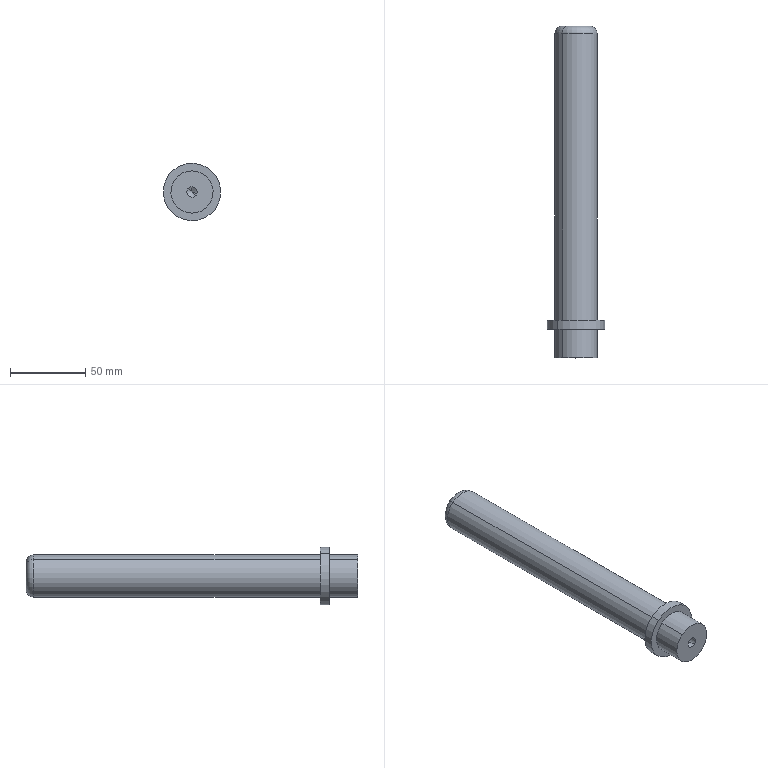Component | SolidWorks | NewDieSet-1_LowerDieSetAssembly-1_GuidePin-2 | 1 solid | 16 faces | box 38 x 220 x 38 mm | volume 137309 mm3 | cylinder 8 | plane 4 | cone 2 | torus 2 | commonest cylinder face diameters 28 x4 6.8 x2 38 x2
build123d program:
from build123d import *

# Parameters (mm, degrees)
SKETCH1_R             = 14
BOSS_EXTRUDE1_DEPTH   = 220
FILLET1_R             = 5
SKETCH4_R             = 19
BOSS_EXTRUDE2_DEPTH   = 6
M8_TAPPED_HOLE1_D     = 6.8
M8_TAPPED_HOLE1_DEPTH = 22.25
M8_TAPPED_HOLE1_TIP   = 2.043


with BuildPart() as part:
    # Sketch1 → Boss-Extrude1 (new body)
    with BuildSketch(Plane.XY):
        Circle(SKETCH1_R)
    extrude(amount=BOSS_EXTRUDE1_DEPTH)

    # Fillet1
    fillet1_edges = [part.edges().sort_by_distance(p)[0] for p in [
        (-14, 0, 0),
    ]]
    fillet(fillet1_edges, radius=FILLET1_R)

    # Sketch4 → Boss-Extrude2 (add)
    with BuildSketch(Plane.XY.offset(201)):
        Circle(SKETCH4_R)
    extrude(amount=-BOSS_EXTRUDE2_DEPTH)

    # M8 Tapped Hole1
    with Locations(Plane.XY.offset(220)):
        with Locations((0, 0)):
            Hole(M8_TAPPED_HOLE1_D / 2, depth=M8_TAPPED_HOLE1_DEPTH)
            with Locations((0, 0, -(M8_TAPPED_HOLE1_DEPTH + M8_TAPPED_HOLE1_TIP / 2))):  # 118° drill point
                Cone(0, M8_TAPPED_HOLE1_D / 2, M8_TAPPED_HOLE1_TIP, mode=Mode.SUBTRACT)


solid = part.part

# Placed as in the assembly
solid = solid.moved(Location((-181.746, 198.927, 138), (90, 0, 0)))
STEP:
#1=COLOUR_RGB('',0.7922,0.8196,0.9333);
#2=FILL_AREA_STYLE_COLOUR('',#1);
#3=FILL_AREA_STYLE('',(#2));
#4=SURFACE_STYLE_FILL_AREA(#3);
#5=SURFACE_SIDE_STYLE('',(#4));
#6=SURFACE_STYLE_USAGE(.BOTH.,#5);
#7=PRESENTATION_STYLE_ASSIGNMENT((#6));
#8=CARTESIAN_POINT('',(-7.241,0.04634,5.536));
#9=VERTEX_POINT('',#8);
#10=CARTESIAN_POINT('',(-7.07,0.04634,5.33));
#11=VERTEX_POINT('',#10);
#12=CARTESIAN_POINT('',(-7.155,0.04634,5.433));
#13=DIRECTION('',(0.,-1.,0.));
#14=DIRECTION('',(0.6389,0.,-0.7693));
#15=AXIS2_PLACEMENT_3D('',#12,#13,#14);
#16=CIRCLE('',#15,0.1339);
#17=EDGE_CURVE('',#9,#11,#16,.T.);
#18=ORIENTED_EDGE('',*,*,#17,.F.);
#19=CARTESIAN_POINT('',(-7.241,-0.8296,5.536));
#20=VERTEX_POINT('',#19);
#21=CARTESIAN_POINT('',(-7.241,-0.8296,5.536));
#22=DIRECTION('',(0.,-1.,0.));
#23=VECTOR('',#22,39.37);
#24=LINE('',#21,#23);
#25=EDGE_CURVE('',#9,#20,#24,.T.);
#26=ORIENTED_EDGE('',*,*,#25,.T.);
#27=CARTESIAN_POINT('',(-7.07,-0.8296,5.33));
#28=VERTEX_POINT('',#27);
#29=CARTESIAN_POINT('',(-7.155,-0.8296,5.433));
#30=DIRECTION('',(0.,-1.,0.));
#31=DIRECTION('',(0.6389,0.,-0.7693));
#32=AXIS2_PLACEMENT_3D('',#29,#30,#31);
#33=CIRCLE('',#32,0.1339);
#34=EDGE_CURVE('',#20,#28,#33,.T.);
#35=ORIENTED_EDGE('',*,*,#34,.T.);
#36=CARTESIAN_POINT('',(-7.07,-0.8296,5.33));
#37=DIRECTION('',(0.,-1.,0.));
#38=VECTOR('',#37,39.37);
#39=LINE('',#36,#38);
#40=EDGE_CURVE('',#11,#28,#39,.T.);
#41=ORIENTED_EDGE('',*,*,#40,.F.);
#42=EDGE_LOOP('',(#18,#26,#35,#41));
#43=FACE_OUTER_BOUND('',#42,.T.);
#44=CARTESIAN_POINT('',(-7.155,-0.8296,5.433));
#45=DIRECTION('',(0.,-1.,0.));
#46=DIRECTION('',(0.6389,0.,-0.7693));
#47=AXIS2_PLACEMENT_3D('',#44,#45,#46);
#48=CYLINDRICAL_SURFACE('',#47,0.1339);
#49=ADVANCED_FACE('',(#43),#48,.F.);
#50=CARTESIAN_POINT('',(-7.155,0.1268,5.433));
#51=VERTEX_POINT('',#50);
#52=CARTESIAN_POINT('',(-7.07,0.04634,5.33));
#53=DIRECTION('',(0.5476,-0.515,-0.6594));
#54=VECTOR('',#53,39.37);
#55=LINE('',#52,#54);
#56=EDGE_CURVE('',#51,#11,#55,.T.);
#57=ORIENTED_EDGE('',*,*,#56,.F.);
#58=CARTESIAN_POINT('',(-7.241,0.04634,5.536));
#59=DIRECTION('',(-0.5476,-0.515,0.6594));
#60=VECTOR('',#59,39.37);
#61=LINE('',#58,#60);
#62=EDGE_CURVE('',#51,#9,#61,.T.);
#63=ORIENTED_EDGE('',*,*,#62,.T.);
#64=ORIENTED_EDGE('',*,*,#17,.T.);
#65=EDGE_LOOP('',(#57,#63,#64));
#66=FACE_OUTER_BOUND('',#65,.T.);
#67=CARTESIAN_POINT('',(-7.155,0.04634,5.433));
#68=DIRECTION('',(0.,-1.,0.));
#69=DIRECTION('',(0.6389,0.,-0.7693));
#70=AXIS2_PLACEMENT_3D('',#67,#68,#69);
#71=CONICAL_SURFACE('',#70,0.1339,1.03);
#72=ADVANCED_FACE('',(#66),#71,.F.);
#73=CARTESIAN_POINT('',(-6.803,-0.8296,5.009));
#74=VERTEX_POINT('',#73);
#75=CARTESIAN_POINT('',(-7.508,-0.8296,5.857));
#76=VERTEX_POINT('',#75);
#77=CARTESIAN_POINT('',(-7.155,-0.8296,5.433));
#78=DIRECTION('',(0.,-1.,0.));
#79=DIRECTION('',(0.6389,0.,-0.7693));
#80=AXIS2_PLACEMENT_3D('',#77,#78,#79);
#81=CIRCLE('',#80,0.5512);
#82=EDGE_CURVE('',#74,#76,#81,.T.);
#83=ORIENTED_EDGE('',*,*,#82,.F.);
#84=CARTESIAN_POINT('',(-6.803,-0.08161,5.009));
#85=VERTEX_POINT('',#84);
#86=CARTESIAN_POINT('',(-6.803,-0.8296,5.009));
#87=DIRECTION('',(0.,1.,0.));
#88=VECTOR('',#87,39.37);
#89=LINE('',#86,#88);
#90=EDGE_CURVE('',#74,#85,#89,.T.);
#91=ORIENTED_EDGE('',*,*,#90,.T.);
#92=CARTESIAN_POINT('',(-7.508,-0.08161,5.857));
#93=VERTEX_POINT('',#92);
#94=CARTESIAN_POINT('',(-7.155,-0.08161,5.433));
#95=DIRECTION('',(0.,-1.,0.));
#96=DIRECTION('',(0.6389,0.,-0.7693));
#97=AXIS2_PLACEMENT_3D('',#94,#95,#96);
#98=CIRCLE('',#97,0.5512);
#99=EDGE_CURVE('',#85,#93,#98,.T.);
#100=ORIENTED_EDGE('',*,*,#99,.T.);
#101=CARTESIAN_POINT('',(-7.508,-0.8296,5.857));
#102=DIRECTION('',(0.,1.,0.));
#103=VECTOR('',#102,39.37);
#104=LINE('',#101,#103);
#105=EDGE_CURVE('',#76,#93,#104,.T.);
#106=ORIENTED_EDGE('',*,*,#105,.F.);
#107=EDGE_LOOP('',(#83,#91,#100,#106));
#108=FACE_OUTER_BOUND('',#107,.T.);
#109=CARTESIAN_POINT('',(-7.155,-0.8296,5.433));
#110=DIRECTION('',(0.,1.,0.));
#111=DIRECTION('',(-0.6389,0.,0.7693));
#112=AXIS2_PLACEMENT_3D('',#109,#110,#111);
#113=CYLINDRICAL_SURFACE('',#112,0.5512);
#114=ADVANCED_FACE('',(#108),#113,.T.);
#115=CARTESIAN_POINT('',(-6.677,0.1546,4.858));
#116=VERTEX_POINT('',#115);
#117=CARTESIAN_POINT('',(-7.633,0.1546,6.009));
#118=VERTEX_POINT('',#117);
#119=CARTESIAN_POINT('',(-7.155,0.1546,5.433));
#120=DIRECTION('',(0.,-1.,0.));
#121=DIRECTION('',(0.6389,0.,-0.7693));
#122=AXIS2_PLACEMENT_3D('',#119,#120,#121);
#123=CIRCLE('',#122,0.748);
#124=EDGE_CURVE('',#116,#118,#123,.T.);
#125=ORIENTED_EDGE('',*,*,#124,.T.);
#126=CARTESIAN_POINT('',(-7.633,-0.08161,6.009));
#127=VERTEX_POINT('',#126);
#128=CARTESIAN_POINT('',(-7.633,0.1546,6.009));
#129=DIRECTION('',(0.,-1.,0.));
#130=VECTOR('',#129,39.37);
#131=LINE('',#128,#130);
#132=EDGE_CURVE('',#118,#127,#131,.T.);
#133=ORIENTED_EDGE('',*,*,#132,.T.);
#134=CARTESIAN_POINT('',(-6.677,-0.08161,4.858));
#135=VERTEX_POINT('',#134);
#136=CARTESIAN_POINT('',(-7.155,-0.08161,5.433));
#137=DIRECTION('',(0.,-1.,0.));
#138=DIRECTION('',(0.6389,0.,-0.7693));
#139=AXIS2_PLACEMENT_3D('',#136,#137,#138);
#140=CIRCLE('',#139,0.748);
#141=EDGE_CURVE('',#135,#127,#140,.T.);
#142=ORIENTED_EDGE('',*,*,#141,.F.);
#143=CARTESIAN_POINT('',(-6.677,0.1546,4.858));
#144=DIRECTION('',(0.,-1.,0.));
#145=VECTOR('',#144,39.37);
#146=LINE('',#143,#145);
#147=EDGE_CURVE('',#116,#135,#146,.T.);
#148=ORIENTED_EDGE('',*,*,#147,.F.);
#149=EDGE_LOOP('',(#125,#133,#142,#148));
#150=FACE_OUTER_BOUND('',#149,.T.);
#151=CARTESIAN_POINT('',(-7.155,0.1546,5.433));
#152=DIRECTION('',(0.,-1.,0.));
#153=DIRECTION('',(0.6389,0.,-0.7693));
#154=AXIS2_PLACEMENT_3D('',#151,#152,#153);
#155=CYLINDRICAL_SURFACE('',#154,0.748);
#156=ADVANCED_FACE('',(#150),#155,.T.);
#157=CARTESIAN_POINT('',(-7.382,7.832,5.706));
#158=VERTEX_POINT('',#157);
#159=CARTESIAN_POINT('',(-6.929,7.832,5.16));
#160=VERTEX_POINT('',#159);
#161=CARTESIAN_POINT('',(-7.155,7.832,5.433));
#162=DIRECTION('',(0.,1.,0.));
#163=DIRECTION('',(0.6389,0.,-0.7693));
#164=AXIS2_PLACEMENT_3D('',#161,#162,#163);
#165=CIRCLE('',#164,0.3543);
#166=EDGE_CURVE('',#158,#160,#165,.T.);
#167=ORIENTED_EDGE('',*,*,#166,.F.);
#168=CARTESIAN_POINT('',(-7.508,7.635,5.857));
#169=VERTEX_POINT('',#168);
#170=CARTESIAN_POINT('',(-7.382,7.635,5.706));
#171=DIRECTION('',(0.7693,0.,0.6389));
#172=DIRECTION('',(0.6389,0.,-0.7693));
#173=AXIS2_PLACEMENT_3D('',#170,#171,#172);
#174=CIRCLE('',#173,0.1969);
#175=EDGE_CURVE('',#158,#169,#174,.T.);
#176=ORIENTED_EDGE('',*,*,#175,.T.);
#177=CARTESIAN_POINT('',(-6.803,7.635,5.009));
#178=VERTEX_POINT('',#177);
#179=CARTESIAN_POINT('',(-7.155,7.635,5.433));
#180=DIRECTION('',(0.,-1.,0.));
#181=DIRECTION('',(0.6389,0.,-0.7693));
#182=AXIS2_PLACEMENT_3D('',#179,#180,#181);
#183=CIRCLE('',#182,0.5512);
#184=EDGE_CURVE('',#178,#169,#183,.T.);
#185=ORIENTED_EDGE('',*,*,#184,.F.);
#186=CARTESIAN_POINT('',(-6.929,7.635,5.16));
#187=DIRECTION('',(-0.7693,0.,-0.6389));
#188=DIRECTION('',(-0.6389,0.,0.7693));
#189=AXIS2_PLACEMENT_3D('',#186,#187,#188);
#190=CIRCLE('',#189,0.1969);
#191=EDGE_CURVE('',#160,#178,#190,.T.);
#192=ORIENTED_EDGE('',*,*,#191,.F.);
#193=EDGE_LOOP('',(#167,#176,#185,#192));
#194=FACE_OUTER_BOUND('',#193,.T.);
#195=CARTESIAN_POINT('',(-7.155,7.635,5.433));
#196=DIRECTION('',(0.,-1.,0.));
#197=DIRECTION('',(0.6389,0.,-0.7693));
#198=AXIS2_PLACEMENT_3D('',#195,#196,#197);
#199=TOROIDAL_SURFACE('',#198,0.3543,0.1969);
#200=ADVANCED_FACE('',(#194),#199,.T.);
#201=CARTESIAN_POINT('',(-6.803,0.1546,5.009));
#202=VERTEX_POINT('',#201);
#203=CARTESIAN_POINT('',(-7.508,0.1546,5.857));
#204=VERTEX_POINT('',#203);
#205=CARTESIAN_POINT('',(-7.155,0.1546,5.433));
#206=DIRECTION('',(0.,-1.,0.));
#207=DIRECTION('',(0.6389,0.,-0.7693));
#208=AXIS2_PLACEMENT_3D('',#205,#206,#207);
#209=CIRCLE('',#208,0.5512);
#210=EDGE_CURVE('',#202,#204,#209,.T.);
#211=ORIENTED_EDGE('',*,*,#210,.F.);
#212=CARTESIAN_POINT('',(-6.803,-0.8296,5.009));
#213=DIRECTION('',(0.,1.,0.));
#214=VECTOR('',#213,39.37);
#215=LINE('',#212,#214);
#216=EDGE_CURVE('',#202,#178,#215,.T.);
#217=ORIENTED_EDGE('',*,*,#216,.T.);
#218=ORIENTED_EDGE('',*,*,#184,.T.);
#219=CARTESIAN_POINT('',(-7.508,-0.8296,5.857));
#220=DIRECTION('',(0.,1.,0.));
#221=VECTOR('',#220,39.37);
#222=LINE('',#219,#221);
#223=EDGE_CURVE('',#204,#169,#222,.T.);
#224=ORIENTED_EDGE('',*,*,#223,.F.);
#225=EDGE_LOOP('',(#211,#217,#218,#224));
#226=FACE_OUTER_BOUND('',#225,.T.);
#227=CARTESIAN_POINT('',(-7.155,-0.8296,5.433));
#228=DIRECTION('',(0.,1.,0.));
#229=DIRECTION('',(-0.6389,0.,0.7693));
#230=AXIS2_PLACEMENT_3D('',#227,#228,#229);
#231=CYLINDRICAL_SURFACE('',#230,0.5512);
#232=ADVANCED_FACE('',(#226),#231,.T.);
#233=ORIENTED_EDGE('',*,*,#216,.F.);
#234=CARTESIAN_POINT('',(-7.155,0.1546,5.433));
#235=DIRECTION('',(0.,-1.,0.));
#236=DIRECTION('',(0.6389,0.,-0.7693));
#237=AXIS2_PLACEMENT_3D('',#234,#235,#236);
#238=CIRCLE('',#237,0.5512);
#239=EDGE_CURVE('',#204,#202,#238,.T.);
#240=ORIENTED_EDGE('',*,*,#239,.F.);
#241=ORIENTED_EDGE('',*,*,#223,.T.);
#242=CARTESIAN_POINT('',(-7.155,7.635,5.433));
#243=DIRECTION('',(0.,-1.,0.));
#244=DIRECTION('',(0.6389,0.,-0.7693));
#245=AXIS2_PLACEMENT_3D('',#242,#243,#244);
#246=CIRCLE('',#245,0.5512);
#247=EDGE_CURVE('',#169,#178,#246,.T.);
#248=ORIENTED_EDGE('',*,*,#247,.T.);
#249=EDGE_LOOP('',(#233,#240,#241,#248));
#250=FACE_OUTER_BOUND('',#249,.T.);
#251=CARTESIAN_POINT('',(-7.155,-0.8296,5.433));
#252=DIRECTION('',(0.,1.,0.));
#253=DIRECTION('',(-0.6389,0.,0.7693));
#254=AXIS2_PLACEMENT_3D('',#251,#252,#253);
#255=CYLINDRICAL_SURFACE('',#254,0.5512);
#256=ADVANCED_FACE('',(#250),#255,.T.);
#257=CARTESIAN_POINT('',(-7.155,7.832,5.433));
#258=DIRECTION('',(0.,1.,0.));
#259=DIRECTION('',(0.6389,0.,-0.7693));
#260=AXIS2_PLACEMENT_3D('',#257,#258,#259);
#261=CIRCLE('',#260,0.3543);
#262=EDGE_CURVE('',#160,#158,#261,.T.);
#263=ORIENTED_EDGE('',*,*,#262,.T.);
#264=ORIENTED_EDGE('',*,*,#166,.T.);
#265=EDGE_LOOP('',(#263,#264));
#266=FACE_OUTER_BOUND('',#265,.T.);
#267=CARTESIAN_POINT('',(-7.155,7.832,5.433));
#268=DIRECTION('',(0.,-1.,0.));
#269=DIRECTION('',(0.6389,0.,-0.7693));
#270=AXIS2_PLACEMENT_3D('',#267,#268,#269);
#271=PLANE('',#270);
#272=ADVANCED_FACE('',(#266),#271,.F.);
#273=ORIENTED_EDGE('',*,*,#175,.F.);
#274=ORIENTED_EDGE('',*,*,#262,.F.);
#275=ORIENTED_EDGE('',*,*,#191,.T.);
#276=ORIENTED_EDGE('',*,*,#247,.F.);
#277=EDGE_LOOP('',(#273,#274,#275,#276));
#278=FACE_OUTER_BOUND('',#277,.T.);
#279=CARTESIAN_POINT('',(-7.155,7.635,5.433));
#280=DIRECTION('',(0.,-1.,0.));
#281=DIRECTION('',(0.6389,0.,-0.7693));
#282=AXIS2_PLACEMENT_3D('',#279,#280,#281);
#283=TOROIDAL_SURFACE('',#282,0.3543,0.1969);
#284=ADVANCED_FACE('',(#278),#283,.T.);
#285=ORIENTED_EDGE('',*,*,#132,.F.);
#286=CARTESIAN_POINT('',(-7.155,0.1546,5.433));
#287=DIRECTION('',(0.,-1.,0.));
#288=DIRECTION('',(0.6389,0.,-0.7693));
#289=AXIS2_PLACEMENT_3D('',#286,#287,#288);
#290=CIRCLE('',#289,0.748);
#291=EDGE_CURVE('',#118,#116,#290,.T.);
#292=ORIENTED_EDGE('',*,*,#291,.T.);
#293=ORIENTED_EDGE('',*,*,#147,.T.);
#294=CARTESIAN_POINT('',(-7.155,-0.08161,5.433));
#295=DIRECTION('',(0.,-1.,0.));
#296=DIRECTION('',(0.6389,0.,-0.7693));
#297=AXIS2_PLACEMENT_3D('',#294,#295,#296);
#298=CIRCLE('',#297,0.748);
#299=EDGE_CURVE('',#127,#135,#298,.T.);
#300=ORIENTED_EDGE('',*,*,#299,.F.);
#301=EDGE_LOOP('',(#285,#292,#293,#300));
#302=FACE_OUTER_BOUND('',#301,.T.);
#303=CARTESIAN_POINT('',(-7.155,0.1546,5.433));
#304=DIRECTION('',(0.,-1.,0.));
#305=DIRECTION('',(0.6389,0.,-0.7693));
#306=AXIS2_PLACEMENT_3D('',#303,#304,#305);
#307=CYLINDRICAL_SURFACE('',#306,0.748);
#308=ADVANCED_FACE('',(#302),#307,.T.);
#309=ORIENTED_EDGE('',*,*,#239,.T.);
#310=ORIENTED_EDGE('',*,*,#210,.T.);
#311=EDGE_LOOP('',(#309,#310));
#312=FACE_BOUND('',#311,.T.);
#313=ORIENTED_EDGE('',*,*,#124,.F.);
#314=ORIENTED_EDGE('',*,*,#291,.F.);
#315=EDGE_LOOP('',(#313,#314));
#316=FACE_OUTER_BOUND('',#315,.T.);
#317=CARTESIAN_POINT('',(-7.155,0.1546,5.433));
#318=DIRECTION('',(0.,-1.,0.));
#319=DIRECTION('',(0.6389,0.,-0.7693));
#320=AXIS2_PLACEMENT_3D('',#317,#318,#319);
#321=PLANE('',#320);
#322=ADVANCED_FACE('',(#312,#316),#321,.F.);
#323=CARTESIAN_POINT('',(-7.155,-0.08161,5.433));
#324=DIRECTION('',(0.,-1.,0.));
#325=DIRECTION('',(0.6389,0.,-0.7693));
#326=AXIS2_PLACEMENT_3D('',#323,#324,#325);
#327=CIRCLE('',#326,0.5512);
#328=EDGE_CURVE('',#93,#85,#327,.T.);
#329=ORIENTED_EDGE('',*,*,#328,.F.);
#330=ORIENTED_EDGE('',*,*,#99,.F.);
#331=EDGE_LOOP('',(#329,#330));
#332=FACE_BOUND('',#331,.T.);
#333=ORIENTED_EDGE('',*,*,#141,.T.);
#334=ORIENTED_EDGE('',*,*,#299,.T.);
#335=EDGE_LOOP('',(#333,#334));
#336=FACE_OUTER_BOUND('',#335,.T.);
#337=CARTESIAN_POINT('',(-7.155,-0.08161,5.433));
#338=DIRECTION('',(0.,-1.,0.));
#339=DIRECTION('',(0.6389,0.,-0.7693));
#340=AXIS2_PLACEMENT_3D('',#337,#338,#339);
#341=PLANE('',#340);
#342=ADVANCED_FACE('',(#332,#336),#341,.T.);
#343=CARTESIAN_POINT('',(-7.155,-0.8296,5.433));
#344=DIRECTION('',(0.,-1.,0.));
#345=DIRECTION('',(0.6389,0.,-0.7693));
#346=AXIS2_PLACEMENT_3D('',#343,#344,#345);
#347=CIRCLE('',#346,0.1339);
#348=EDGE_CURVE('',#28,#20,#347,.T.);
#349=ORIENTED_EDGE('',*,*,#348,.F.);
#350=ORIENTED_EDGE('',*,*,#34,.F.);
#351=EDGE_LOOP('',(#349,#350));
#352=FACE_BOUND('',#351,.T.);
#353=CARTESIAN_POINT('',(-7.155,-0.8296,5.433));
#354=DIRECTION('',(0.,-1.,0.));
#355=DIRECTION('',(0.6389,0.,-0.7693));
#356=AXIS2_PLACEMENT_3D('',#353,#354,#355);
#357=CIRCLE('',#356,0.5512);
#358=EDGE_CURVE('',#76,#74,#357,.T.);
#359=ORIENTED_EDGE('',*,*,#358,.T.);
#360=ORIENTED_EDGE('',*,*,#82,.T.);
#361=EDGE_LOOP('',(#359,#360));
#362=FACE_OUTER_BOUND('',#361,.T.);
#363=CARTESIAN_POINT('',(-7.155,-0.8296,5.433));
#364=DIRECTION('',(0.,-1.,0.));
#365=DIRECTION('',(0.6389,0.,-0.7693));
#366=AXIS2_PLACEMENT_3D('',#363,#364,#365);
#367=PLANE('',#366);
#368=ADVANCED_FACE('',(#352,#362),#367,.T.);
#369=ORIENTED_EDGE('',*,*,#90,.F.);
#370=ORIENTED_EDGE('',*,*,#358,.F.);
#371=ORIENTED_EDGE('',*,*,#105,.T.);
#372=ORIENTED_EDGE('',*,*,#328,.T.);
#373=EDGE_LOOP('',(#369,#370,#371,#372));
#374=FACE_OUTER_BOUND('',#373,.T.);
#375=CARTESIAN_POINT('',(-7.155,-0.8296,5.433));
#376=DIRECTION('',(0.,1.,0.));
#377=DIRECTION('',(-0.6389,0.,0.7693));
#378=AXIS2_PLACEMENT_3D('',#375,#376,#377);
#379=CYLINDRICAL_SURFACE('',#378,0.5512);
#380=ADVANCED_FACE('',(#374),#379,.T.);
#381=ORIENTED_EDGE('',*,*,#62,.F.);
#382=ORIENTED_EDGE('',*,*,#56,.T.);
#383=CARTESIAN_POINT('',(-7.155,0.04634,5.433));
#384=DIRECTION('',(0.,-1.,0.));
#385=DIRECTION('',(0.6389,0.,-0.7693));
#386=AXIS2_PLACEMENT_3D('',#383,#384,#385);
#387=CIRCLE('',#386,0.1339);
#388=EDGE_CURVE('',#11,#9,#387,.T.);
#389=ORIENTED_EDGE('',*,*,#388,.T.);
#390=EDGE_LOOP('',(#381,#382,#389));
#391=FACE_OUTER_BOUND('',#390,.T.);
#392=CARTESIAN_POINT('',(-7.155,0.04634,5.433));
#393=DIRECTION('',(0.,-1.,0.));
#394=DIRECTION('',(0.6389,0.,-0.7693));
#395=AXIS2_PLACEMENT_3D('',#392,#393,#394);
#396=CONICAL_SURFACE('',#395,0.1339,1.03);
#397=ADVANCED_FACE('',(#391),#396,.F.);
#398=ORIENTED_EDGE('',*,*,#25,.F.);
#399=ORIENTED_EDGE('',*,*,#388,.F.);
#400=ORIENTED_EDGE('',*,*,#40,.T.);
#401=ORIENTED_EDGE('',*,*,#348,.T.);
#402=EDGE_LOOP('',(#398,#399,#400,#401));
#403=FACE_OUTER_BOUND('',#402,.T.);
#404=CARTESIAN_POINT('',(-7.155,-0.8296,5.433));
#405=DIRECTION('',(0.,-1.,0.));
#406=DIRECTION('',(0.6389,0.,-0.7693));
#407=AXIS2_PLACEMENT_3D('',#404,#405,#406);
#408=CYLINDRICAL_SURFACE('',#407,0.1339);
#409=ADVANCED_FACE('',(#403),#408,.F.);
#410=CLOSED_SHELL('',(#49,#72,#114,#156,#200,#232,#256,#272,#284,#308,#322,#342,#368,#380,#397,#409));
#411=MANIFOLD_SOLID_BREP('',#410);
#412=STYLED_ITEM('',(#7),#411);
#413=PRESENTATION_LAYER_ASSIGNMENT('','',(#412));
#414=(LENGTH_UNIT()NAMED_UNIT(*)SI_UNIT($,.METRE.));
#415=LENGTH_MEASURE_WITH_UNIT(LENGTH_MEASURE(0.0254),#414);
#416=DIMENSIONAL_EXPONENTS(1.,0.,0.,0.,0.,0.,0.);
#417=(CONVERSION_BASED_UNIT('',#415)LENGTH_UNIT()NAMED_UNIT(#416));
#418=UNCERTAINTY_MEASURE_WITH_UNIT(LENGTH_MEASURE(0.00001),#417,'','');
#419=(NAMED_UNIT(*)PLANE_ANGLE_UNIT()SI_UNIT($,.RADIAN.));
#420=(NAMED_UNIT(*)SI_UNIT($,.STERADIAN.)SOLID_ANGLE_UNIT());
#421=(GEOMETRIC_REPRESENTATION_CONTEXT(3)GLOBAL_UNCERTAINTY_ASSIGNED_CONTEXT((#418))GLOBAL_UNIT_ASSIGNED_CONTEXT((#417,#419,#420))REPRESENTATION_CONTEXT('',''));
#422=MECHANICAL_DESIGN_GEOMETRIC_PRESENTATION_REPRESENTATION('',(#412),#421);
#423=CARTESIAN_POINT('',(0.,0.,0.));
#424=DIRECTION('',(0.,0.,1.));
#425=DIRECTION('',(1.,0.,0.));
#426=AXIS2_PLACEMENT_3D('',#423,#424,#425);
#427=(LENGTH_UNIT()NAMED_UNIT(*)SI_UNIT($,.METRE.));
#428=LENGTH_MEASURE_WITH_UNIT(LENGTH_MEASURE(0.0254),#427);
#429=DIMENSIONAL_EXPONENTS(1.,0.,0.,0.,0.,0.,0.);
#430=(CONVERSION_BASED_UNIT('',#428)LENGTH_UNIT()NAMED_UNIT(#429));
#431=UNCERTAINTY_MEASURE_WITH_UNIT(LENGTH_MEASURE(0.00001),#430,'','');
#432=(NAMED_UNIT(*)PLANE_ANGLE_UNIT()SI_UNIT($,.RADIAN.));
#433=(NAMED_UNIT(*)SI_UNIT($,.STERADIAN.)SOLID_ANGLE_UNIT());
#434=(GEOMETRIC_REPRESENTATION_CONTEXT(3)GLOBAL_UNCERTAINTY_ASSIGNED_CONTEXT((#431))GLOBAL_UNIT_ASSIGNED_CONTEXT((#430,#432,#433))REPRESENTATION_CONTEXT('',''));
#435=ADVANCED_BREP_SHAPE_REPRESENTATION('',(#411,#426),#434);